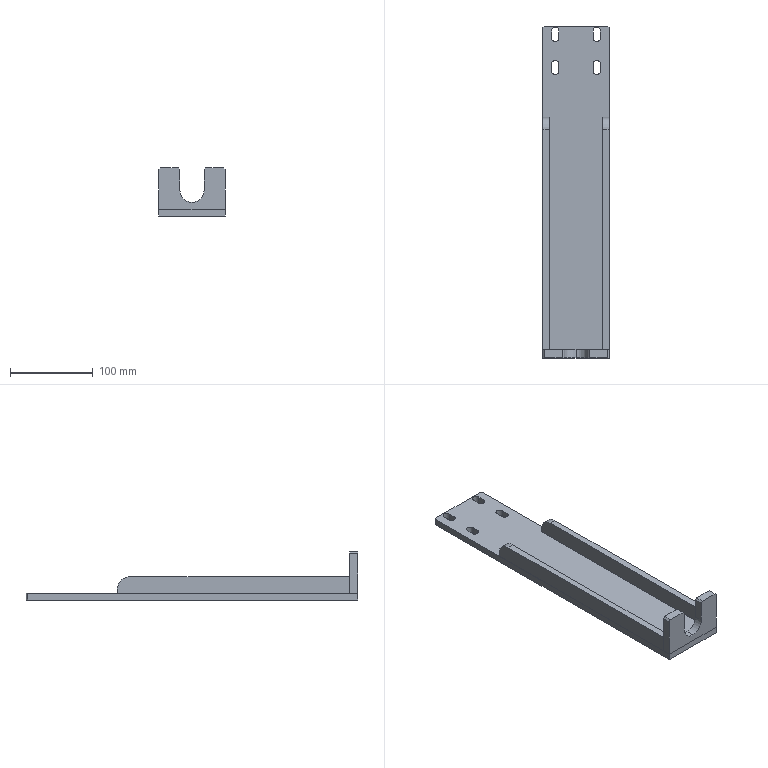Component | SolidWorks | AUTO-SpinDryWashing-01-03000001-1 | 4 solids | 53 faces | box 80 x 400 x 58 mm | volume 369243 mm3 | plane 41 | cylinder 12 | commonest cylinder face diameters 9 x8 29 x2 30 x2 | material AISI 316 Stainless Steel Sheet (SS)
build123d program:
from build123d import *

# Parameters (mm, degrees)
SKETCH1_W             = 80
SKETCH1_H             = 400
BOSS_EXTRUDE1_DEPTH   = 8
SKETCH2_W             = 80
SKETCH2_H             = 10
BOSS_EXTRUDE2_DEPTH   = 50
CUT_EXTRUDE1_DEPTH    = 60
SKETCH4_W             = 8
SKETCH4_H             = 280
BOSS_EXTRUDE3_DEPTH   = 20
BOSS_EXTRUDE3_2_DEPTH = 20
FILLET1_R             = 15
FILLET2_R             = 15
CUT_EXTRUDE2_DEPTH    = 10
LPATTERN1_COUNT       = 2
LPATTERN1_PITCH       = 50
LPATTERN1_COUNT_DIR2  = 2
LPATTERN1_PITCH_DIR2  = 40
CHAMFER1_SIZE         = 2
CHAMFER2_SIZE         = 2


with BuildPart() as part:
    # Sketch1 → Boss-Extrude1 (new body)
    with BuildSketch(Plane.XY):
        with Locations((0, 200)):
            Rectangle(SKETCH1_W, SKETCH1_H)
    extrude(amount=BOSS_EXTRUDE1_DEPTH)

    # Sketch5 → Cut-Extrude2 (cut)
    with BuildSketch(Plane.XY.offset(8)):
        with BuildLine():
            Line((-20.5, 394), (-20.5, 386))
            ThreePointArc((-20.5, 386), (-25, 381.5), (-29.5, 386))
            Line((-29.5, 386), (-29.5, 394))
            ThreePointArc((-29.5, 394), (-25, 398.5), (-20.5, 394))
        make_face()
    cut_extrude2 = extrude(amount=-CUT_EXTRUDE2_DEPTH, mode=Mode.SUBTRACT)

    # LPattern1: Cut-Extrude2 2 × 2
    with Locations(*[(i * LPATTERN1_PITCH, -j * LPATTERN1_PITCH_DIR2, 0) for i in range(LPATTERN1_COUNT) for j in range(LPATTERN1_COUNT_DIR2) if (i, j) != (0, 0)]):
        add(cut_extrude2, mode=Mode.SUBTRACT)

    # Chamfer1
    chamfer1_edges = [part.edges().sort_by_distance(p)[0] for p in [
        (-40, 400, 4),
        (40, 400, 4),
    ]]
    chamfer(chamfer1_edges, length=CHAMFER1_SIZE)


with BuildPart() as body_2:
    # Sketch2 → Boss-Extrude2 (new body)
    with BuildSketch(Plane.XY.offset(8)):
        with Locations((0, 5)):
            Rectangle(SKETCH2_W, SKETCH2_H)
    extrude(amount=BOSS_EXTRUDE2_DEPTH)

    # Sketch3 → Cut-Extrude1 (cut)
    with BuildSketch(Plane.XZ):
        with BuildLine():
            Line((-14.5, 58), (14.5, 58))
            Line((14.5, 58), (14.5, 31))
            ThreePointArc((14.5, 31), (0, 16.5), (-14.5, 31))
            Line((-14.5, 31), (-14.5, 58))
        make_face()
    extrude(amount=-CUT_EXTRUDE1_DEPTH, mode=Mode.SUBTRACT)

    # Chamfer2
    chamfer2_edges = [body_2.edges().sort_by_distance(p)[0] for p in [
        (-40, 5, 58),
        (14.5, 5, 58),
        (-14.5, 5, 58),
        (40, 5, 58),
    ]]
    chamfer(chamfer2_edges, length=CHAMFER2_SIZE)


with BuildPart() as body_3:
    # Sketch4 → Boss-Extrude3 (new body)
    with BuildSketch(Plane.XY.offset(8)):
        with Locations((-36, 150)):
            Rectangle(SKETCH4_W, SKETCH4_H)
    extrude(amount=BOSS_EXTRUDE3_DEPTH)

    # Fillet2
    fillet2_edges = [body_3.edges().sort_by_distance(p)[0] for p in [
        (-36, 290, 28),
    ]]
    fillet(fillet2_edges, radius=FILLET2_R)


with BuildPart() as body_4:
    # Sketch4 → Boss-Extrude3 2 (new body)
    with BuildSketch(Plane.XY.offset(8)):
        with Locations((36, 150)):
            Rectangle(SKETCH4_W, SKETCH4_H)
    extrude(amount=BOSS_EXTRUDE3_2_DEPTH)

    # Fillet1
    fillet1_edges = [body_4.edges().sort_by_distance(p)[0] for p in [
        (36, 290, 28),
    ]]
    fillet(fillet1_edges, radius=FILLET1_R)


solid = Compound([part.part, body_2.part, body_3.part, body_4.part])